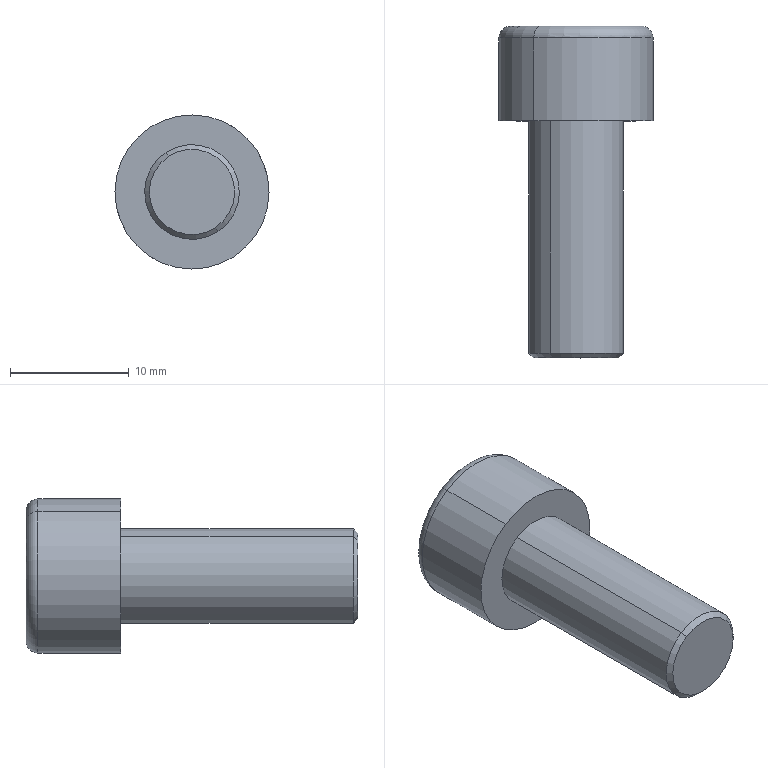Component | SolidWorks | hexagon socket head cap screws gb-21 | 1 solid | 25 faces | box 13 x 28 x 13 mm | volume 1916 mm3 | plane 15 | cone 4 | cylinder 4 | torus 2 | commonest cylinder face diameters 8 x2 13 x2
STEP:
#1=CARTESIAN_POINT('',(-5.134,31.204,20.214));
#2=VERTEX_POINT('',#1);
#3=CARTESIAN_POINT('',(-5.289,31.204,20.451));
#4=VERTEX_POINT('',#3);
#5=CARTESIAN_POINT('',(-5.211,31.204,20.332));
#6=DIRECTION('',(0.,-1.,0.));
#7=DIRECTION('',(0.5469,0.,-0.8372));
#8=AXIS2_PLACEMENT_3D('',#5,#6,#7);
#9=CIRCLE('',#8,0.1417);
#10=EDGE_CURVE('',#2,#4,#9,.T.);
#11=ORIENTED_EDGE('',*,*,#10,.F.);
#12=CARTESIAN_POINT('',(-5.125,31.22,20.2));
#13=VERTEX_POINT('',#12);
#14=CARTESIAN_POINT('',(-5.134,31.204,20.214));
#15=DIRECTION('',(0.3867,0.7071,-0.592));
#16=VECTOR('',#15,39.37);
#17=LINE('',#14,#16);
#18=EDGE_CURVE('',#2,#13,#17,.T.);
#19=ORIENTED_EDGE('',*,*,#18,.T.);
#20=CARTESIAN_POINT('',(-5.297,31.22,20.464));
#21=VERTEX_POINT('',#20);
#22=CARTESIAN_POINT('',(-5.211,31.22,20.332));
#23=DIRECTION('',(-0.,1.,-0.));
#24=DIRECTION('',(0.5469,0.,-0.8372));
#25=AXIS2_PLACEMENT_3D('',#22,#23,#24);
#26=CIRCLE('',#25,0.1575);
#27=EDGE_CURVE('',#21,#13,#26,.T.);
#28=ORIENTED_EDGE('',*,*,#27,.F.);
#29=CARTESIAN_POINT('',(-5.289,31.204,20.451));
#30=DIRECTION('',(-0.3867,0.7071,0.592));
#31=VECTOR('',#30,39.37);
#32=LINE('',#29,#31);
#33=EDGE_CURVE('',#4,#21,#32,.T.);
#34=ORIENTED_EDGE('',*,*,#33,.F.);
#35=EDGE_LOOP('',(#11,#19,#28,#34));
#36=FACE_OUTER_BOUND('',#35,.T.);
#37=CARTESIAN_POINT('',(-5.211,31.204,20.332));
#38=DIRECTION('',(-0.,1.,-0.));
#39=DIRECTION('',(-0.5469,0.,0.8372));
#40=AXIS2_PLACEMENT_3D('',#37,#38,#39);
#41=CONICAL_SURFACE('',#40,0.1417,0.7854);
#42=ADVANCED_FACE('',(#36),#41,.T.);
#43=CARTESIAN_POINT('',(-5.33,32.306,20.514));
#44=VERTEX_POINT('',#43);
#45=CARTESIAN_POINT('',(-5.093,32.306,20.151));
#46=VERTEX_POINT('',#45);
#47=CARTESIAN_POINT('',(-5.211,32.306,20.332));
#48=DIRECTION('',(-0.,1.,-0.));
#49=DIRECTION('',(0.5469,0.,-0.8372));
#50=AXIS2_PLACEMENT_3D('',#47,#48,#49);
#51=CIRCLE('',#50,0.2165);
#52=EDGE_CURVE('',#44,#46,#51,.T.);
#53=ORIENTED_EDGE('',*,*,#52,.F.);
#54=CARTESIAN_POINT('',(-5.351,32.267,20.547));
#55=VERTEX_POINT('',#54);
#56=CARTESIAN_POINT('',(-5.33,32.267,20.514));
#57=DIRECTION('',(0.8372,0.,0.5469));
#58=DIRECTION('',(0.5469,0.,-0.8372));
#59=AXIS2_PLACEMENT_3D('',#56,#57,#58);
#60=CIRCLE('',#59,0.03937);
#61=EDGE_CURVE('',#44,#55,#60,.T.);
#62=ORIENTED_EDGE('',*,*,#61,.T.);
#63=CARTESIAN_POINT('',(-5.071,32.267,20.118));
#64=VERTEX_POINT('',#63);
#65=CARTESIAN_POINT('',(-5.211,32.267,20.332));
#66=DIRECTION('',(0.,-1.,0.));
#67=DIRECTION('',(0.5469,0.,-0.8372));
#68=AXIS2_PLACEMENT_3D('',#65,#66,#67);
#69=CIRCLE('',#68,0.2559);
#70=EDGE_CURVE('',#64,#55,#69,.T.);
#71=ORIENTED_EDGE('',*,*,#70,.F.);
#72=CARTESIAN_POINT('',(-5.093,32.267,20.151));
#73=DIRECTION('',(-0.8372,-0.,-0.5469));
#74=DIRECTION('',(-0.5469,0.,0.8372));
#75=AXIS2_PLACEMENT_3D('',#72,#73,#74);
#76=CIRCLE('',#75,0.03937);
#77=EDGE_CURVE('',#46,#64,#76,.T.);
#78=ORIENTED_EDGE('',*,*,#77,.F.);
#79=EDGE_LOOP('',(#53,#62,#71,#78));
#80=FACE_OUTER_BOUND('',#79,.T.);
#81=CARTESIAN_POINT('',(-5.211,32.267,20.332));
#82=DIRECTION('',(0.,-1.,0.));
#83=DIRECTION('',(0.5469,0.,-0.8372));
#84=AXIS2_PLACEMENT_3D('',#81,#82,#83);
#85=TOROIDAL_SURFACE('',#84,0.2165,0.03937);
#86=ADVANCED_FACE('',(#80),#85,.T.);
#87=CARTESIAN_POINT('',(-5.211,32.081,20.332));
#88=VERTEX_POINT('',#87);
#89=CARTESIAN_POINT('',(-5.276,32.149,20.431));
#90=VERTEX_POINT('',#89);
#91=CARTESIAN_POINT('',(-5.276,32.149,20.431));
#92=DIRECTION('',(-0.4737,0.5,0.725));
#93=VECTOR('',#92,39.37);
#94=LINE('',#91,#93);
#95=EDGE_CURVE('',#88,#90,#94,.T.);
#96=ORIENTED_EDGE('',*,*,#95,.F.);
#97=CARTESIAN_POINT('',(-5.147,32.149,20.233));
#98=VERTEX_POINT('',#97);
#99=CARTESIAN_POINT('',(-5.147,32.149,20.233));
#100=DIRECTION('',(0.4737,0.5,-0.725));
#101=VECTOR('',#100,39.37);
#102=LINE('',#99,#101);
#103=EDGE_CURVE('',#88,#98,#102,.T.);
#104=ORIENTED_EDGE('',*,*,#103,.T.);
#105=CARTESIAN_POINT('',(-5.205,32.149,20.214));
#106=VERTEX_POINT('',#105);
#107=CARTESIAN_POINT('',(-5.211,32.149,20.332));
#108=DIRECTION('',(0.,-1.,0.));
#109=DIRECTION('',(-0.5469,0.,0.8372));
#110=AXIS2_PLACEMENT_3D('',#107,#108,#109);
#111=CIRCLE('',#110,0.1181);
#112=EDGE_CURVE('',#106,#98,#111,.T.);
#113=ORIENTED_EDGE('',*,*,#112,.F.);
#114=CARTESIAN_POINT('',(-5.31,32.149,20.268));
#115=VERTEX_POINT('',#114);
#116=CARTESIAN_POINT('',(-5.211,32.149,20.332));
#117=DIRECTION('',(0.,-1.,0.));
#118=DIRECTION('',(-0.5469,0.,0.8372));
#119=AXIS2_PLACEMENT_3D('',#116,#117,#118);
#120=CIRCLE('',#119,0.1181);
#121=EDGE_CURVE('',#115,#106,#120,.T.);
#122=ORIENTED_EDGE('',*,*,#121,.F.);
#123=CARTESIAN_POINT('',(-5.317,32.149,20.386));
#124=VERTEX_POINT('',#123);
#125=CARTESIAN_POINT('',(-5.211,32.149,20.332));
#126=DIRECTION('',(0.,-1.,0.));
#127=DIRECTION('',(-0.5469,0.,0.8372));
#128=AXIS2_PLACEMENT_3D('',#125,#126,#127);
#129=CIRCLE('',#128,0.1181);
#130=EDGE_CURVE('',#124,#115,#129,.T.);
#131=ORIENTED_EDGE('',*,*,#130,.F.);
#132=CARTESIAN_POINT('',(-5.211,32.149,20.332));
#133=DIRECTION('',(0.,-1.,0.));
#134=DIRECTION('',(-0.5469,0.,0.8372));
#135=AXIS2_PLACEMENT_3D('',#132,#133,#134);
#136=CIRCLE('',#135,0.1181);
#137=EDGE_CURVE('',#90,#124,#136,.T.);
#138=ORIENTED_EDGE('',*,*,#137,.F.);
#139=EDGE_LOOP('',(#96,#104,#113,#122,#131,#138));
#140=FACE_OUTER_BOUND('',#139,.T.);
#141=CARTESIAN_POINT('',(-5.211,32.149,20.332));
#142=DIRECTION('',(-0.,1.,-0.));
#143=DIRECTION('',(-0.5469,0.,0.8372));
#144=AXIS2_PLACEMENT_3D('',#141,#142,#143);
#145=CONICAL_SURFACE('',#144,0.1181,1.047);
#146=ADVANCED_FACE('',(#140),#145,.F.);
#147=ORIENTED_EDGE('',*,*,#27,.T.);
#148=CARTESIAN_POINT('',(-5.125,31.991,20.2));
#149=VERTEX_POINT('',#148);
#150=CARTESIAN_POINT('',(-5.125,31.204,20.2));
#151=DIRECTION('',(-0.,1.,-0.));
#152=VECTOR('',#151,39.37);
#153=LINE('',#150,#152);
#154=EDGE_CURVE('',#13,#149,#153,.T.);
#155=ORIENTED_EDGE('',*,*,#154,.T.);
#156=CARTESIAN_POINT('',(-5.297,31.991,20.464));
#157=VERTEX_POINT('',#156);
#158=CARTESIAN_POINT('',(-5.211,31.991,20.332));
#159=DIRECTION('',(0.,-1.,0.));
#160=DIRECTION('',(0.5469,0.,-0.8372));
#161=AXIS2_PLACEMENT_3D('',#158,#159,#160);
#162=CIRCLE('',#161,0.1575);
#163=EDGE_CURVE('',#149,#157,#162,.T.);
#164=ORIENTED_EDGE('',*,*,#163,.T.);
#165=CARTESIAN_POINT('',(-5.297,31.204,20.464));
#166=DIRECTION('',(-0.,1.,-0.));
#167=VECTOR('',#166,39.37);
#168=LINE('',#165,#167);
#169=EDGE_CURVE('',#21,#157,#168,.T.);
#170=ORIENTED_EDGE('',*,*,#169,.F.);
#171=EDGE_LOOP('',(#147,#155,#164,#170));
#172=FACE_OUTER_BOUND('',#171,.T.);
#173=CARTESIAN_POINT('',(-5.211,31.204,20.332));
#174=DIRECTION('',(-0.,1.,-0.));
#175=DIRECTION('',(-0.5469,0.,0.8372));
#176=AXIS2_PLACEMENT_3D('',#173,#174,#175);
#177=CYLINDRICAL_SURFACE('',#176,0.1575);
#178=ADVANCED_FACE('',(#172),#177,.T.);
#179=CARTESIAN_POINT('',(-5.071,31.991,20.118));
#180=VERTEX_POINT('',#179);
#181=CARTESIAN_POINT('',(-5.351,31.991,20.547));
#182=VERTEX_POINT('',#181);
#183=CARTESIAN_POINT('',(-5.211,31.991,20.332));
#184=DIRECTION('',(0.,-1.,0.));
#185=DIRECTION('',(0.5469,0.,-0.8372));
#186=AXIS2_PLACEMENT_3D('',#183,#184,#185);
#187=CIRCLE('',#186,0.2559);
#188=EDGE_CURVE('',#180,#182,#187,.T.);
#189=ORIENTED_EDGE('',*,*,#188,.F.);
#190=CARTESIAN_POINT('',(-5.071,31.991,20.118));
#191=DIRECTION('',(-0.,1.,-0.));
#192=VECTOR('',#191,39.37);
#193=LINE('',#190,#192);
#194=EDGE_CURVE('',#180,#64,#193,.T.);
#195=ORIENTED_EDGE('',*,*,#194,.T.);
#196=ORIENTED_EDGE('',*,*,#70,.T.);
#197=CARTESIAN_POINT('',(-5.351,31.991,20.547));
#198=DIRECTION('',(-0.,1.,-0.));
#199=VECTOR('',#198,39.37);
#200=LINE('',#197,#199);
#201=EDGE_CURVE('',#182,#55,#200,.T.);
#202=ORIENTED_EDGE('',*,*,#201,.F.);
#203=EDGE_LOOP('',(#189,#195,#196,#202));
#204=FACE_OUTER_BOUND('',#203,.T.);
#205=CARTESIAN_POINT('',(-5.211,31.991,20.332));
#206=DIRECTION('',(-0.,1.,-0.));
#207=DIRECTION('',(-0.5469,0.,0.8372));
#208=AXIS2_PLACEMENT_3D('',#205,#206,#207);
#209=CYLINDRICAL_SURFACE('',#208,0.2559);
#210=ADVANCED_FACE('',(#204),#209,.T.);
#211=CARTESIAN_POINT('',(-5.347,32.149,20.325));
#212=VERTEX_POINT('',#211);
#213=CARTESIAN_POINT('',(-5.286,32.149,20.446));
#214=DIRECTION('',(-0.4515,-0.,-0.8923));
#215=VECTOR('',#214,39.37);
#216=LINE('',#213,#215);
#217=EDGE_CURVE('',#124,#212,#216,.T.);
#218=ORIENTED_EDGE('',*,*,#217,.F.);
#219=ORIENTED_EDGE('',*,*,#130,.T.);
#220=CARTESIAN_POINT('',(-5.347,32.149,20.325));
#221=DIRECTION('',(0.5469,0.,-0.8372));
#222=VECTOR('',#221,39.37);
#223=LINE('',#220,#222);
#224=EDGE_CURVE('',#212,#115,#223,.T.);
#225=ORIENTED_EDGE('',*,*,#224,.F.);
#226=EDGE_LOOP('',(#218,#219,#225));
#227=FACE_OUTER_BOUND('',#226,.T.);
#228=CARTESIAN_POINT('',(-5.409,32.149,20.203));
#229=DIRECTION('',(-0.,1.,-0.));
#230=DIRECTION('',(-0.5469,-0.,0.8372));
#231=AXIS2_PLACEMENT_3D('',#228,#229,#230);
#232=PLANE('',#231);
#233=ADVANCED_FACE('',(#227),#232,.T.);
#234=CARTESIAN_POINT('',(-5.273,32.149,20.211));
#235=VERTEX_POINT('',#234);
#236=CARTESIAN_POINT('',(-5.347,32.149,20.325));
#237=DIRECTION('',(0.5469,0.,-0.8372));
#238=VECTOR('',#237,39.37);
#239=LINE('',#236,#238);
#240=EDGE_CURVE('',#115,#235,#239,.T.);
#241=ORIENTED_EDGE('',*,*,#240,.F.);
#242=ORIENTED_EDGE('',*,*,#121,.T.);
#243=CARTESIAN_POINT('',(-5.273,32.149,20.211));
#244=DIRECTION('',(0.9985,0.,0.05508));
#245=VECTOR('',#244,39.37);
#246=LINE('',#243,#245);
#247=EDGE_CURVE('',#235,#106,#246,.T.);
#248=ORIENTED_EDGE('',*,*,#247,.F.);
#249=EDGE_LOOP('',(#241,#242,#248));
#250=FACE_OUTER_BOUND('',#249,.T.);
#251=CARTESIAN_POINT('',(-5.409,32.149,20.203));
#252=DIRECTION('',(-0.,1.,-0.));
#253=DIRECTION('',(-0.5469,-0.,0.8372));
#254=AXIS2_PLACEMENT_3D('',#251,#252,#253);
#255=PLANE('',#254);
#256=ADVANCED_FACE('',(#250),#255,.T.);
#257=CARTESIAN_POINT('',(-5.137,32.149,20.218));
#258=VERTEX_POINT('',#257);
#259=CARTESIAN_POINT('',(-5.273,32.149,20.211));
#260=DIRECTION('',(0.9985,0.,0.05508));
#261=VECTOR('',#260,39.37);
#262=LINE('',#259,#261);
#263=EDGE_CURVE('',#106,#258,#262,.T.);
#264=ORIENTED_EDGE('',*,*,#263,.F.);
#265=ORIENTED_EDGE('',*,*,#112,.T.);
#266=CARTESIAN_POINT('',(-5.106,32.149,20.279));
#267=VERTEX_POINT('',#266);
#268=CARTESIAN_POINT('',(-5.211,32.149,20.332));
#269=DIRECTION('',(0.,-1.,0.));
#270=DIRECTION('',(-0.5469,0.,0.8372));
#271=AXIS2_PLACEMENT_3D('',#268,#269,#270);
#272=CIRCLE('',#271,0.1181);
#273=EDGE_CURVE('',#98,#267,#272,.T.);
#274=ORIENTED_EDGE('',*,*,#273,.T.);
#275=CARTESIAN_POINT('',(-5.137,32.149,20.218));
#276=DIRECTION('',(0.4515,0.,0.8923));
#277=VECTOR('',#276,39.37);
#278=LINE('',#275,#277);
#279=EDGE_CURVE('',#258,#267,#278,.T.);
#280=ORIENTED_EDGE('',*,*,#279,.F.);
#281=EDGE_LOOP('',(#264,#265,#274,#280));
#282=FACE_OUTER_BOUND('',#281,.T.);
#283=CARTESIAN_POINT('',(-5.409,32.149,20.203));
#284=DIRECTION('',(-0.,1.,-0.));
#285=DIRECTION('',(-0.5469,-0.,0.8372));
#286=AXIS2_PLACEMENT_3D('',#283,#284,#285);
#287=PLANE('',#286);
#288=ADVANCED_FACE('',(#282),#287,.T.);
#289=CARTESIAN_POINT('',(-5.075,32.149,20.34));
#290=VERTEX_POINT('',#289);
#291=CARTESIAN_POINT('',(-5.137,32.149,20.218));
#292=DIRECTION('',(0.4515,0.,0.8923));
#293=VECTOR('',#292,39.37);
#294=LINE('',#291,#293);
#295=EDGE_CURVE('',#267,#290,#294,.T.);
#296=ORIENTED_EDGE('',*,*,#295,.F.);
#297=CARTESIAN_POINT('',(-5.112,32.149,20.397));
#298=VERTEX_POINT('',#297);
#299=CARTESIAN_POINT('',(-5.211,32.149,20.332));
#300=DIRECTION('',(0.,-1.,0.));
#301=DIRECTION('',(0.5469,0.,-0.8372));
#302=AXIS2_PLACEMENT_3D('',#299,#300,#301);
#303=CIRCLE('',#302,0.1181);
#304=EDGE_CURVE('',#267,#298,#303,.T.);
#305=ORIENTED_EDGE('',*,*,#304,.T.);
#306=CARTESIAN_POINT('',(-5.075,32.149,20.34));
#307=DIRECTION('',(-0.5469,-0.,0.8372));
#308=VECTOR('',#307,39.37);
#309=LINE('',#306,#308);
#310=EDGE_CURVE('',#290,#298,#309,.T.);
#311=ORIENTED_EDGE('',*,*,#310,.F.);
#312=EDGE_LOOP('',(#296,#305,#311));
#313=FACE_OUTER_BOUND('',#312,.T.);
#314=CARTESIAN_POINT('',(-5.409,32.149,20.203));
#315=DIRECTION('',(-0.,1.,-0.));
#316=DIRECTION('',(-0.5469,-0.,0.8372));
#317=AXIS2_PLACEMENT_3D('',#314,#315,#316);
#318=PLANE('',#317);
#319=ADVANCED_FACE('',(#313),#318,.T.);
#320=CARTESIAN_POINT('',(-5.15,32.149,20.454));
#321=VERTEX_POINT('',#320);
#322=CARTESIAN_POINT('',(-5.075,32.149,20.34));
#323=DIRECTION('',(-0.5469,-0.,0.8372));
#324=VECTOR('',#323,39.37);
#325=LINE('',#322,#324);
#326=EDGE_CURVE('',#298,#321,#325,.T.);
#327=ORIENTED_EDGE('',*,*,#326,.F.);
#328=CARTESIAN_POINT('',(-5.218,32.149,20.45));
#329=VERTEX_POINT('',#328);
#330=CARTESIAN_POINT('',(-5.211,32.149,20.332));
#331=DIRECTION('',(0.,-1.,0.));
#332=DIRECTION('',(-0.5469,0.,0.8372));
#333=AXIS2_PLACEMENT_3D('',#330,#331,#332);
#334=CIRCLE('',#333,0.1181);
#335=EDGE_CURVE('',#298,#329,#334,.T.);
#336=ORIENTED_EDGE('',*,*,#335,.T.);
#337=CARTESIAN_POINT('',(-5.15,32.149,20.454));
#338=DIRECTION('',(-0.9985,-0.,-0.05508));
#339=VECTOR('',#338,39.37);
#340=LINE('',#337,#339);
#341=EDGE_CURVE('',#321,#329,#340,.T.);
#342=ORIENTED_EDGE('',*,*,#341,.F.);
#343=EDGE_LOOP('',(#327,#336,#342));
#344=FACE_OUTER_BOUND('',#343,.T.);
#345=CARTESIAN_POINT('',(-5.409,32.149,20.203));
#346=DIRECTION('',(-0.,1.,-0.));
#347=DIRECTION('',(-0.5469,-0.,0.8372));
#348=AXIS2_PLACEMENT_3D('',#345,#346,#347);
#349=PLANE('',#348);
#350=ADVANCED_FACE('',(#344),#349,.T.);
#351=CARTESIAN_POINT('',(-5.286,32.149,20.446));
#352=VERTEX_POINT('',#351);
#353=CARTESIAN_POINT('',(-5.15,32.149,20.454));
#354=DIRECTION('',(-0.9985,-0.,-0.05508));
#355=VECTOR('',#354,39.37);
#356=LINE('',#353,#355);
#357=EDGE_CURVE('',#329,#352,#356,.T.);
#358=ORIENTED_EDGE('',*,*,#357,.F.);
#359=CARTESIAN_POINT('',(-5.211,32.149,20.332));
#360=DIRECTION('',(0.,-1.,0.));
#361=DIRECTION('',(-0.5469,0.,0.8372));
#362=AXIS2_PLACEMENT_3D('',#359,#360,#361);
#363=CIRCLE('',#362,0.1181);
#364=EDGE_CURVE('',#329,#90,#363,.T.);
#365=ORIENTED_EDGE('',*,*,#364,.T.);
#366=ORIENTED_EDGE('',*,*,#137,.T.);
#367=CARTESIAN_POINT('',(-5.286,32.149,20.446));
#368=DIRECTION('',(-0.4515,-0.,-0.8923));
#369=VECTOR('',#368,39.37);
#370=LINE('',#367,#369);
#371=EDGE_CURVE('',#352,#124,#370,.T.);
#372=ORIENTED_EDGE('',*,*,#371,.F.);
#373=EDGE_LOOP('',(#358,#365,#366,#372));
#374=FACE_OUTER_BOUND('',#373,.T.);
#375=CARTESIAN_POINT('',(-5.409,32.149,20.203));
#376=DIRECTION('',(-0.,1.,-0.));
#377=DIRECTION('',(-0.5469,-0.,0.8372));
#378=AXIS2_PLACEMENT_3D('',#375,#376,#377);
#379=PLANE('',#378);
#380=ADVANCED_FACE('',(#374),#379,.T.);
#381=CARTESIAN_POINT('',(-5.211,32.306,20.332));
#382=DIRECTION('',(-0.,1.,-0.));
#383=DIRECTION('',(0.5469,0.,-0.8372));
#384=AXIS2_PLACEMENT_3D('',#381,#382,#383);
#385=CIRCLE('',#384,0.2165);
#386=EDGE_CURVE('',#46,#44,#385,.T.);
#387=ORIENTED_EDGE('',*,*,#386,.T.);
#388=ORIENTED_EDGE('',*,*,#52,.T.);
#389=EDGE_LOOP('',(#387,#388));
#390=FACE_OUTER_BOUND('',#389,.T.);
#391=CARTESIAN_POINT('',(-5.273,32.306,20.211));
#392=VERTEX_POINT('',#391);
#393=CARTESIAN_POINT('',(-5.137,32.306,20.218));
#394=VERTEX_POINT('',#393);
#395=CARTESIAN_POINT('',(-5.273,32.306,20.211));
#396=DIRECTION('',(0.9985,0.,0.05508));
#397=VECTOR('',#396,39.37);
#398=LINE('',#395,#397);
#399=EDGE_CURVE('',#392,#394,#398,.T.);
#400=ORIENTED_EDGE('',*,*,#399,.T.);
#401=CARTESIAN_POINT('',(-5.075,32.306,20.34));
#402=VERTEX_POINT('',#401);
#403=CARTESIAN_POINT('',(-5.137,32.306,20.218));
#404=DIRECTION('',(0.4515,0.,0.8923));
#405=VECTOR('',#404,39.37);
#406=LINE('',#403,#405);
#407=EDGE_CURVE('',#394,#402,#406,.T.);
#408=ORIENTED_EDGE('',*,*,#407,.T.);
#409=CARTESIAN_POINT('',(-5.15,32.306,20.454));
#410=VERTEX_POINT('',#409);
#411=CARTESIAN_POINT('',(-5.075,32.306,20.34));
#412=DIRECTION('',(-0.5469,-0.,0.8372));
#413=VECTOR('',#412,39.37);
#414=LINE('',#411,#413);
#415=EDGE_CURVE('',#402,#410,#414,.T.);
#416=ORIENTED_EDGE('',*,*,#415,.T.);
#417=CARTESIAN_POINT('',(-5.286,32.306,20.446));
#418=VERTEX_POINT('',#417);
#419=CARTESIAN_POINT('',(-5.15,32.306,20.454));
#420=DIRECTION('',(-0.9985,-0.,-0.05508));
#421=VECTOR('',#420,39.37);
#422=LINE('',#419,#421);
#423=EDGE_CURVE('',#410,#418,#422,.T.);
#424=ORIENTED_EDGE('',*,*,#423,.T.);
#425=CARTESIAN_POINT('',(-5.347,32.306,20.325));
#426=VERTEX_POINT('',#425);
#427=CARTESIAN_POINT('',(-5.286,32.306,20.446));
#428=DIRECTION('',(-0.4515,-0.,-0.8923));
#429=VECTOR('',#428,39.37);
#430=LINE('',#427,#429);
#431=EDGE_CURVE('',#418,#426,#430,.T.);
#432=ORIENTED_EDGE('',*,*,#431,.T.);
#433=CARTESIAN_POINT('',(-5.347,32.306,20.325));
#434=DIRECTION('',(0.5469,0.,-0.8372));
#435=VECTOR('',#434,39.37);
#436=LINE('',#433,#435);
#437=EDGE_CURVE('',#426,#392,#436,.T.);
#438=ORIENTED_EDGE('',*,*,#437,.T.);
#439=EDGE_LOOP('',(#400,#408,#416,#424,#432,#438));
#440=FACE_BOUND('',#439,.T.);
#441=CARTESIAN_POINT('',(-5.211,32.306,20.332));
#442=DIRECTION('',(0.,-1.,0.));
#443=DIRECTION('',(0.5469,0.,-0.8372));
#444=AXIS2_PLACEMENT_3D('',#441,#442,#443);
#445=PLANE('',#444);
#446=ADVANCED_FACE('',(#390,#440),#445,.F.);
#447=CARTESIAN_POINT('',(-5.211,31.991,20.332));
#448=DIRECTION('',(0.,-1.,0.));
#449=DIRECTION('',(0.5469,0.,-0.8372));
#450=AXIS2_PLACEMENT_3D('',#447,#448,#449);
#451=CIRCLE('',#450,0.2559);
#452=EDGE_CURVE('',#182,#180,#451,.T.);
#453=ORIENTED_EDGE('',*,*,#452,.T.);
#454=ORIENTED_EDGE('',*,*,#188,.T.);
#455=EDGE_LOOP('',(#453,#454));
#456=FACE_OUTER_BOUND('',#455,.T.);
#457=CARTESIAN_POINT('',(-5.211,31.991,20.332));
#458=DIRECTION('',(0.,-1.,0.));
#459=DIRECTION('',(0.5469,0.,-0.8372));
#460=AXIS2_PLACEMENT_3D('',#457,#458,#459);
#461=CIRCLE('',#460,0.1575);
#462=EDGE_CURVE('',#157,#149,#461,.T.);
#463=ORIENTED_EDGE('',*,*,#462,.F.);
#464=ORIENTED_EDGE('',*,*,#163,.F.);
#465=EDGE_LOOP('',(#463,#464));
#466=FACE_BOUND('',#465,.T.);
#467=CARTESIAN_POINT('',(-5.211,31.991,20.332));
#468=DIRECTION('',(0.,-1.,0.));
#469=DIRECTION('',(0.5469,0.,-0.8372));
#470=AXIS2_PLACEMENT_3D('',#467,#468,#469);
#471=PLANE('',#470);
#472=ADVANCED_FACE('',(#456,#466),#471,.T.);
#473=ORIENTED_EDGE('',*,*,#194,.F.);
#474=ORIENTED_EDGE('',*,*,#452,.F.);
#475=ORIENTED_EDGE('',*,*,#201,.T.);
#476=CARTESIAN_POINT('',(-5.211,32.267,20.332));
#477=DIRECTION('',(0.,-1.,0.));
#478=DIRECTION('',(0.5469,0.,-0.8372));
#479=AXIS2_PLACEMENT_3D('',#476,#477,#478);
#480=CIRCLE('',#479,0.2559);
#481=EDGE_CURVE('',#55,#64,#480,.T.);
#482=ORIENTED_EDGE('',*,*,#481,.T.);
#483=EDGE_LOOP('',(#473,#474,#475,#482));
#484=FACE_OUTER_BOUND('',#483,.T.);
#485=CARTESIAN_POINT('',(-5.211,31.991,20.332));
#486=DIRECTION('',(-0.,1.,-0.));
#487=DIRECTION('',(-0.5469,0.,0.8372));
#488=AXIS2_PLACEMENT_3D('',#485,#486,#487);
#489=CYLINDRICAL_SURFACE('',#488,0.2559);
#490=ADVANCED_FACE('',(#484),#489,.T.);
#491=ORIENTED_EDGE('',*,*,#154,.F.);
#492=CARTESIAN_POINT('',(-5.211,31.22,20.332));
#493=DIRECTION('',(-0.,1.,-0.));
#494=DIRECTION('',(0.5469,0.,-0.8372));
#495=AXIS2_PLACEMENT_3D('',#492,#493,#494);
#496=CIRCLE('',#495,0.1575);
#497=EDGE_CURVE('',#13,#21,#496,.T.);
#498=ORIENTED_EDGE('',*,*,#497,.T.);
#499=ORIENTED_EDGE('',*,*,#169,.T.);
#500=ORIENTED_EDGE('',*,*,#462,.T.);
#501=EDGE_LOOP('',(#491,#498,#499,#500));
#502=FACE_OUTER_BOUND('',#501,.T.);
#503=CARTESIAN_POINT('',(-5.211,31.204,20.332));
#504=DIRECTION('',(-0.,1.,-0.));
#505=DIRECTION('',(-0.5469,0.,0.8372));
#506=AXIS2_PLACEMENT_3D('',#503,#504,#505);
#507=CYLINDRICAL_SURFACE('',#506,0.1575);
#508=ADVANCED_FACE('',(#502),#507,.T.);
#509=CARTESIAN_POINT('',(-5.211,31.204,20.332));
#510=DIRECTION('',(0.,-1.,0.));
#511=DIRECTION('',(0.5469,0.,-0.8372));
#512=AXIS2_PLACEMENT_3D('',#509,#510,#511);
#513=CIRCLE('',#512,0.1417);
#514=EDGE_CURVE('',#4,#2,#513,.T.);
#515=ORIENTED_EDGE('',*,*,#514,.T.);
#516=ORIENTED_EDGE('',*,*,#10,.T.);
#517=EDGE_LOOP('',(#515,#516));
#518=FACE_OUTER_BOUND('',#517,.T.);
#519=CARTESIAN_POINT('',(-5.211,31.204,20.332));
#520=DIRECTION('',(0.,-1.,0.));
#521=DIRECTION('',(0.5469,0.,-0.8372));
#522=AXIS2_PLACEMENT_3D('',#519,#520,#521);
#523=PLANE('',#522);
#524=ADVANCED_FACE('',(#518),#523,.T.);
#525=ORIENTED_EDGE('',*,*,#399,.F.);
#526=CARTESIAN_POINT('',(-5.273,32.149,20.211));
#527=DIRECTION('',(-0.,1.,-0.));
#528=VECTOR('',#527,39.37);
#529=LINE('',#526,#528);
#530=EDGE_CURVE('',#235,#392,#529,.T.);
#531=ORIENTED_EDGE('',*,*,#530,.F.);
#532=ORIENTED_EDGE('',*,*,#247,.T.);
#533=ORIENTED_EDGE('',*,*,#263,.T.);
#534=CARTESIAN_POINT('',(-5.137,32.149,20.218));
#535=DIRECTION('',(-0.,1.,-0.));
#536=VECTOR('',#535,39.37);
#537=LINE('',#534,#536);
#538=EDGE_CURVE('',#258,#394,#537,.T.);
#539=ORIENTED_EDGE('',*,*,#538,.T.);
#540=EDGE_LOOP('',(#525,#531,#532,#533,#539));
#541=FACE_OUTER_BOUND('',#540,.T.);
#542=CARTESIAN_POINT('',(-5.273,32.149,20.211));
#543=DIRECTION('',(-0.05508,0.,0.9985));
#544=DIRECTION('',(-0.9985,-0.,-0.05508));
#545=AXIS2_PLACEMENT_3D('',#542,#543,#544);
#546=PLANE('',#545);
#547=ADVANCED_FACE('',(#541),#546,.T.);
#548=ORIENTED_EDGE('',*,*,#407,.F.);
#549=ORIENTED_EDGE('',*,*,#538,.F.);
#550=ORIENTED_EDGE('',*,*,#279,.T.);
#551=ORIENTED_EDGE('',*,*,#295,.T.);
#552=CARTESIAN_POINT('',(-5.075,32.149,20.34));
#553=DIRECTION('',(-0.,1.,-0.));
#554=VECTOR('',#553,39.37);
#555=LINE('',#552,#554);
#556=EDGE_CURVE('',#290,#402,#555,.T.);
#557=ORIENTED_EDGE('',*,*,#556,.T.);
#558=EDGE_LOOP('',(#548,#549,#550,#551,#557));
#559=FACE_OUTER_BOUND('',#558,.T.);
#560=CARTESIAN_POINT('',(-5.137,32.149,20.218));
#561=DIRECTION('',(-0.8923,-0.,0.4515));
#562=DIRECTION('',(-0.4515,-0.,-0.8923));
#563=AXIS2_PLACEMENT_3D('',#560,#561,#562);
#564=PLANE('',#563);
#565=ADVANCED_FACE('',(#559),#564,.T.);
#566=ORIENTED_EDGE('',*,*,#415,.F.);
#567=ORIENTED_EDGE('',*,*,#556,.F.);
#568=ORIENTED_EDGE('',*,*,#310,.T.);
#569=ORIENTED_EDGE('',*,*,#326,.T.);
#570=CARTESIAN_POINT('',(-5.15,32.149,20.454));
#571=DIRECTION('',(-0.,1.,-0.));
#572=VECTOR('',#571,39.37);
#573=LINE('',#570,#572);
#574=EDGE_CURVE('',#321,#410,#573,.T.);
#575=ORIENTED_EDGE('',*,*,#574,.T.);
#576=EDGE_LOOP('',(#566,#567,#568,#569,#575));
#577=FACE_OUTER_BOUND('',#576,.T.);
#578=CARTESIAN_POINT('',(-5.075,32.149,20.34));
#579=DIRECTION('',(-0.8372,-0.,-0.5469));
#580=DIRECTION('',(0.5469,0.,-0.8372));
#581=AXIS2_PLACEMENT_3D('',#578,#579,#580);
#582=PLANE('',#581);
#583=ADVANCED_FACE('',(#577),#582,.T.);
#584=ORIENTED_EDGE('',*,*,#423,.F.);
#585=ORIENTED_EDGE('',*,*,#574,.F.);
#586=ORIENTED_EDGE('',*,*,#341,.T.);
#587=ORIENTED_EDGE('',*,*,#357,.T.);
#588=CARTESIAN_POINT('',(-5.286,32.149,20.446));
#589=DIRECTION('',(-0.,1.,-0.));
#590=VECTOR('',#589,39.37);
#591=LINE('',#588,#590);
#592=EDGE_CURVE('',#352,#418,#591,.T.);
#593=ORIENTED_EDGE('',*,*,#592,.T.);
#594=EDGE_LOOP('',(#584,#585,#586,#587,#593));
#595=FACE_OUTER_BOUND('',#594,.T.);
#596=CARTESIAN_POINT('',(-5.15,32.149,20.454));
#597=DIRECTION('',(0.05508,-0.,-0.9985));
#598=DIRECTION('',(0.9985,0.,0.05508));
#599=AXIS2_PLACEMENT_3D('',#596,#597,#598);
#600=PLANE('',#599);
#601=ADVANCED_FACE('',(#595),#600,.T.);
#602=ORIENTED_EDGE('',*,*,#431,.F.);
#603=ORIENTED_EDGE('',*,*,#592,.F.);
#604=ORIENTED_EDGE('',*,*,#371,.T.);
#605=ORIENTED_EDGE('',*,*,#217,.T.);
#606=CARTESIAN_POINT('',(-5.347,32.149,20.325));
#607=DIRECTION('',(-0.,1.,-0.));
#608=VECTOR('',#607,39.37);
#609=LINE('',#606,#608);
#610=EDGE_CURVE('',#212,#426,#609,.T.);
#611=ORIENTED_EDGE('',*,*,#610,.T.);
#612=EDGE_LOOP('',(#602,#603,#604,#605,#611));
#613=FACE_OUTER_BOUND('',#612,.T.);
#614=CARTESIAN_POINT('',(-5.286,32.149,20.446));
#615=DIRECTION('',(0.8923,0.,-0.4515));
#616=DIRECTION('',(0.4515,0.,0.8923));
#617=AXIS2_PLACEMENT_3D('',#614,#615,#616);
#618=PLANE('',#617);
#619=ADVANCED_FACE('',(#613),#618,.T.);
#620=ORIENTED_EDGE('',*,*,#437,.F.);
#621=ORIENTED_EDGE('',*,*,#610,.F.);
#622=ORIENTED_EDGE('',*,*,#224,.T.);
#623=ORIENTED_EDGE('',*,*,#240,.T.);
#624=ORIENTED_EDGE('',*,*,#530,.T.);
#625=EDGE_LOOP('',(#620,#621,#622,#623,#624));
#626=FACE_OUTER_BOUND('',#625,.T.);
#627=CARTESIAN_POINT('',(-5.347,32.149,20.325));
#628=DIRECTION('',(0.8372,0.,0.5469));
#629=DIRECTION('',(-0.5469,-0.,0.8372));
#630=AXIS2_PLACEMENT_3D('',#627,#628,#629);
#631=PLANE('',#630);
#632=ADVANCED_FACE('',(#626),#631,.T.);
#633=ORIENTED_EDGE('',*,*,#103,.F.);
#634=ORIENTED_EDGE('',*,*,#95,.T.);
#635=ORIENTED_EDGE('',*,*,#364,.F.);
#636=ORIENTED_EDGE('',*,*,#335,.F.);
#637=ORIENTED_EDGE('',*,*,#304,.F.);
#638=ORIENTED_EDGE('',*,*,#273,.F.);
#639=EDGE_LOOP('',(#633,#634,#635,#636,#637,#638));
#640=FACE_OUTER_BOUND('',#639,.T.);
#641=CARTESIAN_POINT('',(-5.211,32.149,20.332));
#642=DIRECTION('',(-0.,1.,-0.));
#643=DIRECTION('',(-0.5469,0.,0.8372));
#644=AXIS2_PLACEMENT_3D('',#641,#642,#643);
#645=CONICAL_SURFACE('',#644,0.1181,1.047);
#646=ADVANCED_FACE('',(#640),#645,.F.);
#647=ORIENTED_EDGE('',*,*,#61,.F.);
#648=ORIENTED_EDGE('',*,*,#386,.F.);
#649=ORIENTED_EDGE('',*,*,#77,.T.);
#650=ORIENTED_EDGE('',*,*,#481,.F.);
#651=EDGE_LOOP('',(#647,#648,#649,#650));
#652=FACE_OUTER_BOUND('',#651,.T.);
#653=CARTESIAN_POINT('',(-5.211,32.267,20.332));
#654=DIRECTION('',(0.,-1.,0.));
#655=DIRECTION('',(0.5469,0.,-0.8372));
#656=AXIS2_PLACEMENT_3D('',#653,#654,#655);
#657=TOROIDAL_SURFACE('',#656,0.2165,0.03937);
#658=ADVANCED_FACE('',(#652),#657,.T.);
#659=ORIENTED_EDGE('',*,*,#18,.F.);
#660=ORIENTED_EDGE('',*,*,#514,.F.);
#661=ORIENTED_EDGE('',*,*,#33,.T.);
#662=ORIENTED_EDGE('',*,*,#497,.F.);
#663=EDGE_LOOP('',(#659,#660,#661,#662));
#664=FACE_OUTER_BOUND('',#663,.T.);
#665=CARTESIAN_POINT('',(-5.211,31.204,20.332));
#666=DIRECTION('',(-0.,1.,-0.));
#667=DIRECTION('',(-0.5469,0.,0.8372));
#668=AXIS2_PLACEMENT_3D('',#665,#666,#667);
#669=CONICAL_SURFACE('',#668,0.1417,0.7854);
#670=ADVANCED_FACE('',(#664),#669,.T.);
#671=CLOSED_SHELL('',(#42,#86,#146,#178,#210,#233,#256,#288,#319,#350,#380,#446,#472,#490,#508,#524,#547,#565,#583,#601,#619,#632,#646,#658,#670));
#672=MANIFOLD_SOLID_BREP('',#671);
#673=CARTESIAN_POINT('',(0.,0.,0.));
#674=DIRECTION('',(0.,0.,1.));
#675=DIRECTION('',(1.,0.,0.));
#676=AXIS2_PLACEMENT_3D('',#673,#674,#675);
#677=(LENGTH_UNIT()NAMED_UNIT(*)SI_UNIT($,.METRE.));
#678=LENGTH_MEASURE_WITH_UNIT(LENGTH_MEASURE(0.0254),#677);
#679=DIMENSIONAL_EXPONENTS(1.,0.,0.,0.,0.,0.,0.);
#680=(CONVERSION_BASED_UNIT('',#678)LENGTH_UNIT()NAMED_UNIT(#679));
#681=UNCERTAINTY_MEASURE_WITH_UNIT(LENGTH_MEASURE(0.00001),#680,'','');
#682=(NAMED_UNIT(*)PLANE_ANGLE_UNIT()SI_UNIT($,.RADIAN.));
#683=(NAMED_UNIT(*)SI_UNIT($,.STERADIAN.)SOLID_ANGLE_UNIT());
#684=(GEOMETRIC_REPRESENTATION_CONTEXT(3)GLOBAL_UNCERTAINTY_ASSIGNED_CONTEXT((#681))GLOBAL_UNIT_ASSIGNED_CONTEXT((#680,#682,#683))REPRESENTATION_CONTEXT('',''));
#685=ADVANCED_BREP_SHAPE_REPRESENTATION('',(#672,#676),#684);
#686=COLOUR_RGB('',0.7922,0.8196,0.9333);
#687=FILL_AREA_STYLE_COLOUR('',#686);
#688=FILL_AREA_STYLE('',(#687));
#689=SURFACE_STYLE_FILL_AREA(#688);
#690=SURFACE_SIDE_STYLE('',(#689));
#691=SURFACE_STYLE_USAGE(.BOTH.,#690);
#692=PRESENTATION_STYLE_ASSIGNMENT((#691));
#693=STYLED_ITEM('',(#692),#672);
#694=PRESENTATION_LAYER_ASSIGNMENT('','',(#693));
#695=(LENGTH_UNIT()NAMED_UNIT(*)SI_UNIT($,.METRE.));
#696=LENGTH_MEASURE_WITH_UNIT(LENGTH_MEASURE(0.0254),#695);
#697=DIMENSIONAL_EXPONENTS(1.,0.,0.,0.,0.,0.,0.);
#698=(CONVERSION_BASED_UNIT('',#696)LENGTH_UNIT()NAMED_UNIT(#697));
#699=UNCERTAINTY_MEASURE_WITH_UNIT(LENGTH_MEASURE(0.00001),#698,'','');
#700=(NAMED_UNIT(*)PLANE_ANGLE_UNIT()SI_UNIT($,.RADIAN.));
#701=(NAMED_UNIT(*)SI_UNIT($,.STERADIAN.)SOLID_ANGLE_UNIT());
#702=(GEOMETRIC_REPRESENTATION_CONTEXT(3)GLOBAL_UNCERTAINTY_ASSIGNED_CONTEXT((#699))GLOBAL_UNIT_ASSIGNED_CONTEXT((#698,#700,#701))REPRESENTATION_CONTEXT('',''));
#703=MECHANICAL_DESIGN_GEOMETRIC_PRESENTATION_REPRESENTATION('',(#693),#702);